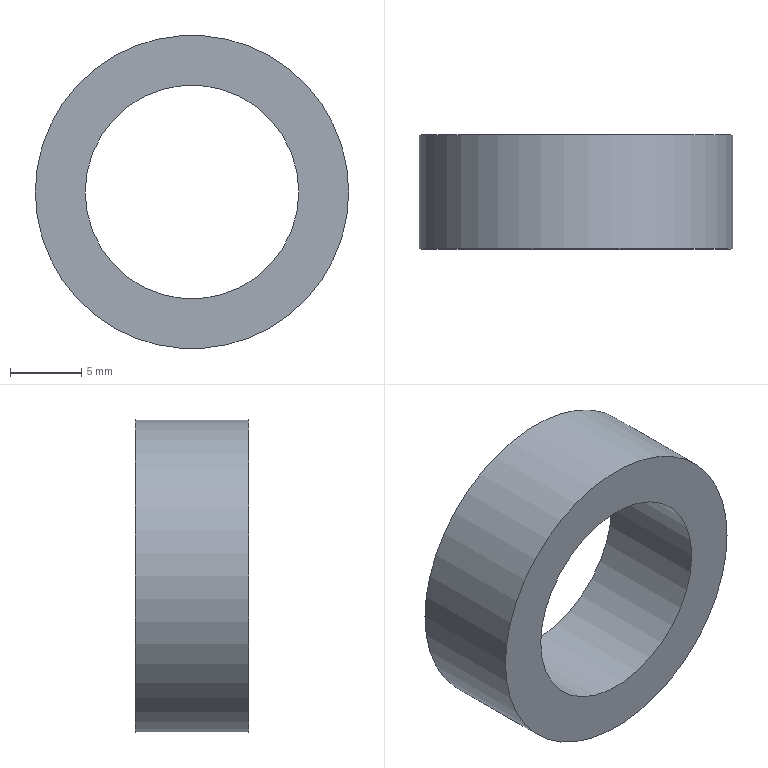Component | NX | 8_2 | 1 solid | 4 faces | box 22 x 8 x 22 mm | volume 1627 mm3 | cylinder 2 | plane 2 | commonest cylinder face diameters 22 x1 15 x1
STEP:
#1=CARTESIAN_POINT('',(0.,0.,0.));
#2=DIRECTION('',(0.,0.,1.));
#3=DIRECTION('',(1.,0.,0.));
#4=AXIS2_PLACEMENT_3D('',#1,#2,#3);
#5=CARTESIAN_POINT('',(6.42,30.798,-0.));
#6=VERTEX_POINT('',#5);
#7=CARTESIAN_POINT('',(-4.58,30.798,0.));
#8=DIRECTION('',(0.,-1.,0.));
#9=DIRECTION('',(1.,0.,-0.));
#10=AXIS2_PLACEMENT_3D('',#7,#8,#9);
#11=CIRCLE('',#10,11.);
#12=CARTESIAN_POINT('',(-4.58,30.798,0.));
#13=DIRECTION('',(0.,-1.,0.));
#14=DIRECTION('',(-1.,0.,0.));
#15=AXIS2_PLACEMENT_3D('',#12,#13,#14);
#16=CYLINDRICAL_SURFACE('',#15,11.);
#17=CARTESIAN_POINT('',(3.142,0.));
#18=DIRECTION('',(1.,0.));
#19=VECTOR('',#18,1.);
#20=LINE('',#17,#19);
#21=(GEOMETRIC_REPRESENTATION_CONTEXT(2)PARAMETRIC_REPRESENTATION_CONTEXT()REPRESENTATION_CONTEXT('',''));
#22=DEFINITIONAL_REPRESENTATION('',(#20),#21);
#23=PCURVE('',#16,#22);
#24=CARTESIAN_POINT('',(-4.58,30.798,0.));
#25=DIRECTION('',(0.,-1.,0.));
#26=DIRECTION('',(-1.,0.,0.));
#27=AXIS2_PLACEMENT_3D('',#24,#25,#26);
#28=PLANE('',#27);
#29=CARTESIAN_POINT('',(0.,0.));
#30=DIRECTION('',(-1.,0.));
#31=AXIS2_PLACEMENT_2D('',#29,#30);
#32=CIRCLE('',#31,11.);
#33=(GEOMETRIC_REPRESENTATION_CONTEXT(2)PARAMETRIC_REPRESENTATION_CONTEXT()REPRESENTATION_CONTEXT('',''));
#34=DEFINITIONAL_REPRESENTATION('',(#32),#33);
#35=PCURVE('',#28,#34);
#36=SURFACE_CURVE('',#11,(#23,#35),.PCURVE_S1.);
#37=EDGE_CURVE('',#6,#6,#36,.T.);
#38=ORIENTED_EDGE('',*,*,#37,.T.);
#39=CARTESIAN_POINT('',(6.42,22.798,-0.));
#40=VERTEX_POINT('',#39);
#41=CARTESIAN_POINT('',(6.42,30.798,-0.));
#42=CARTESIAN_POINT('',(6.42,22.798,-0.));
#43=B_SPLINE_CURVE_WITH_KNOTS('',1,(#41,#42),.UNSPECIFIED.,.F.,.F.,(2,2),(0.,8.),.PIECEWISE_BEZIER_KNOTS.);
#44=CARTESIAN_POINT('',(9.425,0.));
#45=DIRECTION('',(0.,1.));
#46=VECTOR('',#45,1.);
#47=LINE('',#44,#46);
#48=(GEOMETRIC_REPRESENTATION_CONTEXT(2)PARAMETRIC_REPRESENTATION_CONTEXT()REPRESENTATION_CONTEXT('',''));
#49=DEFINITIONAL_REPRESENTATION('',(#47),#48);
#50=PCURVE('',#16,#49);
#51=CARTESIAN_POINT('',(3.142,0.));
#52=DIRECTION('',(0.,1.));
#53=VECTOR('',#52,1.);
#54=LINE('',#51,#53);
#55=(GEOMETRIC_REPRESENTATION_CONTEXT(2)PARAMETRIC_REPRESENTATION_CONTEXT()REPRESENTATION_CONTEXT('',''));
#56=DEFINITIONAL_REPRESENTATION('',(#54),#55);
#57=PCURVE('',#16,#56);
#58=SEAM_CURVE('',#43,(#50,#57),.PCURVE_S1.);
#59=EDGE_CURVE('',#6,#40,#58,.T.);
#60=ORIENTED_EDGE('',*,*,#59,.T.);
#61=CARTESIAN_POINT('',(-4.58,22.798,0.));
#62=DIRECTION('',(0.,-1.,0.));
#63=DIRECTION('',(1.,0.,-0.));
#64=AXIS2_PLACEMENT_3D('',#61,#62,#63);
#65=CIRCLE('',#64,11.);
#66=CARTESIAN_POINT('',(3.142,8.));
#67=DIRECTION('',(1.,0.));
#68=VECTOR('',#67,1.);
#69=LINE('',#66,#68);
#70=(GEOMETRIC_REPRESENTATION_CONTEXT(2)PARAMETRIC_REPRESENTATION_CONTEXT()REPRESENTATION_CONTEXT('',''));
#71=DEFINITIONAL_REPRESENTATION('',(#69),#70);
#72=PCURVE('',#16,#71);
#73=CARTESIAN_POINT('',(-4.58,22.798,0.));
#74=DIRECTION('',(0.,-1.,0.));
#75=DIRECTION('',(-1.,0.,0.));
#76=AXIS2_PLACEMENT_3D('',#73,#74,#75);
#77=PLANE('',#76);
#78=CARTESIAN_POINT('',(0.,0.));
#79=DIRECTION('',(-1.,0.));
#80=AXIS2_PLACEMENT_2D('',#78,#79);
#81=CIRCLE('',#80,11.);
#82=(GEOMETRIC_REPRESENTATION_CONTEXT(2)PARAMETRIC_REPRESENTATION_CONTEXT()REPRESENTATION_CONTEXT('',''));
#83=DEFINITIONAL_REPRESENTATION('',(#81),#82);
#84=PCURVE('',#77,#83);
#85=SURFACE_CURVE('',#65,(#72,#84),.PCURVE_S1.);
#86=EDGE_CURVE('',#40,#40,#85,.T.);
#87=ORIENTED_EDGE('',*,*,#86,.F.);
#88=ORIENTED_EDGE('',*,*,#59,.F.);
#89=EDGE_LOOP('',(#38,#60,#87,#88));
#90=FACE_BOUND('',#89,.T.);
#91=ADVANCED_FACE('',(#90),#16,.T.);
#92=CARTESIAN_POINT('',(2.92,30.798,-0.));
#93=VERTEX_POINT('',#92);
#94=CARTESIAN_POINT('',(-4.58,30.798,0.));
#95=DIRECTION('',(0.,-1.,0.));
#96=DIRECTION('',(1.,0.,-0.));
#97=AXIS2_PLACEMENT_3D('',#94,#95,#96);
#98=CIRCLE('',#97,7.5);
#99=CARTESIAN_POINT('',(-4.58,30.798,0.));
#100=DIRECTION('',(0.,-1.,0.));
#101=DIRECTION('',(-1.,0.,0.));
#102=AXIS2_PLACEMENT_3D('',#99,#100,#101);
#103=CYLINDRICAL_SURFACE('',#102,7.5);
#104=CARTESIAN_POINT('',(3.142,0.));
#105=DIRECTION('',(1.,0.));
#106=VECTOR('',#105,1.);
#107=LINE('',#104,#106);
#108=(GEOMETRIC_REPRESENTATION_CONTEXT(2)PARAMETRIC_REPRESENTATION_CONTEXT()REPRESENTATION_CONTEXT('',''));
#109=DEFINITIONAL_REPRESENTATION('',(#107),#108);
#110=PCURVE('',#103,#109);
#111=CARTESIAN_POINT('',(0.,0.));
#112=DIRECTION('',(-1.,0.));
#113=AXIS2_PLACEMENT_2D('',#111,#112);
#114=CIRCLE('',#113,7.5);
#115=(GEOMETRIC_REPRESENTATION_CONTEXT(2)PARAMETRIC_REPRESENTATION_CONTEXT()REPRESENTATION_CONTEXT('',''));
#116=DEFINITIONAL_REPRESENTATION('',(#114),#115);
#117=PCURVE('',#28,#116);
#118=SURFACE_CURVE('',#98,(#110,#117),.PCURVE_S1.);
#119=EDGE_CURVE('',#93,#93,#118,.T.);
#120=ORIENTED_EDGE('',*,*,#119,.T.);
#121=CARTESIAN_POINT('',(2.92,22.798,-0.));
#122=VERTEX_POINT('',#121);
#123=CARTESIAN_POINT('',(2.92,30.798,-0.));
#124=CARTESIAN_POINT('',(2.92,22.798,-0.));
#125=B_SPLINE_CURVE_WITH_KNOTS('',1,(#123,#124),.UNSPECIFIED.,.F.,.F.,(2,2),(0.,8.),.PIECEWISE_BEZIER_KNOTS.);
#126=CARTESIAN_POINT('',(9.425,0.));
#127=DIRECTION('',(0.,1.));
#128=VECTOR('',#127,1.);
#129=LINE('',#126,#128);
#130=(GEOMETRIC_REPRESENTATION_CONTEXT(2)PARAMETRIC_REPRESENTATION_CONTEXT()REPRESENTATION_CONTEXT('',''));
#131=DEFINITIONAL_REPRESENTATION('',(#129),#130);
#132=PCURVE('',#103,#131);
#133=CARTESIAN_POINT('',(3.142,0.));
#134=DIRECTION('',(0.,1.));
#135=VECTOR('',#134,1.);
#136=LINE('',#133,#135);
#137=(GEOMETRIC_REPRESENTATION_CONTEXT(2)PARAMETRIC_REPRESENTATION_CONTEXT()REPRESENTATION_CONTEXT('',''));
#138=DEFINITIONAL_REPRESENTATION('',(#136),#137);
#139=PCURVE('',#103,#138);
#140=SEAM_CURVE('',#125,(#132,#139),.PCURVE_S1.);
#141=EDGE_CURVE('',#93,#122,#140,.T.);
#142=ORIENTED_EDGE('',*,*,#141,.T.);
#143=CARTESIAN_POINT('',(-4.58,22.798,0.));
#144=DIRECTION('',(0.,-1.,0.));
#145=DIRECTION('',(1.,0.,-0.));
#146=AXIS2_PLACEMENT_3D('',#143,#144,#145);
#147=CIRCLE('',#146,7.5);
#148=CARTESIAN_POINT('',(3.142,8.));
#149=DIRECTION('',(1.,0.));
#150=VECTOR('',#149,1.);
#151=LINE('',#148,#150);
#152=(GEOMETRIC_REPRESENTATION_CONTEXT(2)PARAMETRIC_REPRESENTATION_CONTEXT()REPRESENTATION_CONTEXT('',''));
#153=DEFINITIONAL_REPRESENTATION('',(#151),#152);
#154=PCURVE('',#103,#153);
#155=CARTESIAN_POINT('',(0.,0.));
#156=DIRECTION('',(-1.,0.));
#157=AXIS2_PLACEMENT_2D('',#155,#156);
#158=CIRCLE('',#157,7.5);
#159=(GEOMETRIC_REPRESENTATION_CONTEXT(2)PARAMETRIC_REPRESENTATION_CONTEXT()REPRESENTATION_CONTEXT('',''));
#160=DEFINITIONAL_REPRESENTATION('',(#158),#159);
#161=PCURVE('',#77,#160);
#162=SURFACE_CURVE('',#147,(#154,#161),.PCURVE_S1.);
#163=EDGE_CURVE('',#122,#122,#162,.T.);
#164=ORIENTED_EDGE('',*,*,#163,.F.);
#165=ORIENTED_EDGE('',*,*,#141,.F.);
#166=EDGE_LOOP('',(#120,#142,#164,#165));
#167=FACE_BOUND('',#166,.F.);
#168=ADVANCED_FACE('',(#167),#103,.F.);
#169=ORIENTED_EDGE('',*,*,#37,.F.);
#170=EDGE_LOOP('',(#169));
#171=FACE_BOUND('',#170,.T.);
#172=ORIENTED_EDGE('',*,*,#119,.T.);
#173=EDGE_LOOP('',(#172));
#174=FACE_BOUND('',#173,.T.);
#175=ADVANCED_FACE('',(#171,#174),#28,.F.);
#176=ORIENTED_EDGE('',*,*,#86,.T.);
#177=EDGE_LOOP('',(#176));
#178=FACE_BOUND('',#177,.T.);
#179=ORIENTED_EDGE('',*,*,#163,.F.);
#180=EDGE_LOOP('',(#179));
#181=FACE_BOUND('',#180,.T.);
#182=ADVANCED_FACE('',(#178,#181),#77,.T.);
#183=CLOSED_SHELL('',(#91,#168,#175,#182));
#184=MANIFOLD_SOLID_BREP('',#183);
#185=(LENGTH_UNIT()NAMED_UNIT(*)SI_UNIT(.MILLI.,.METRE.));
#186=UNCERTAINTY_MEASURE_WITH_UNIT(LENGTH_MEASURE(0.00001),#185,'','');
#187=(NAMED_UNIT(*)PLANE_ANGLE_UNIT()SI_UNIT($,.RADIAN.));
#188=(NAMED_UNIT(*)SI_UNIT($,.STERADIAN.)SOLID_ANGLE_UNIT());
#189=(GEOMETRIC_REPRESENTATION_CONTEXT(3)GLOBAL_UNCERTAINTY_ASSIGNED_CONTEXT((#186))GLOBAL_UNIT_ASSIGNED_CONTEXT((#185,#187,#188))REPRESENTATION_CONTEXT('',''));
#190=ADVANCED_BREP_SHAPE_REPRESENTATION('',(#4,#184),#189);